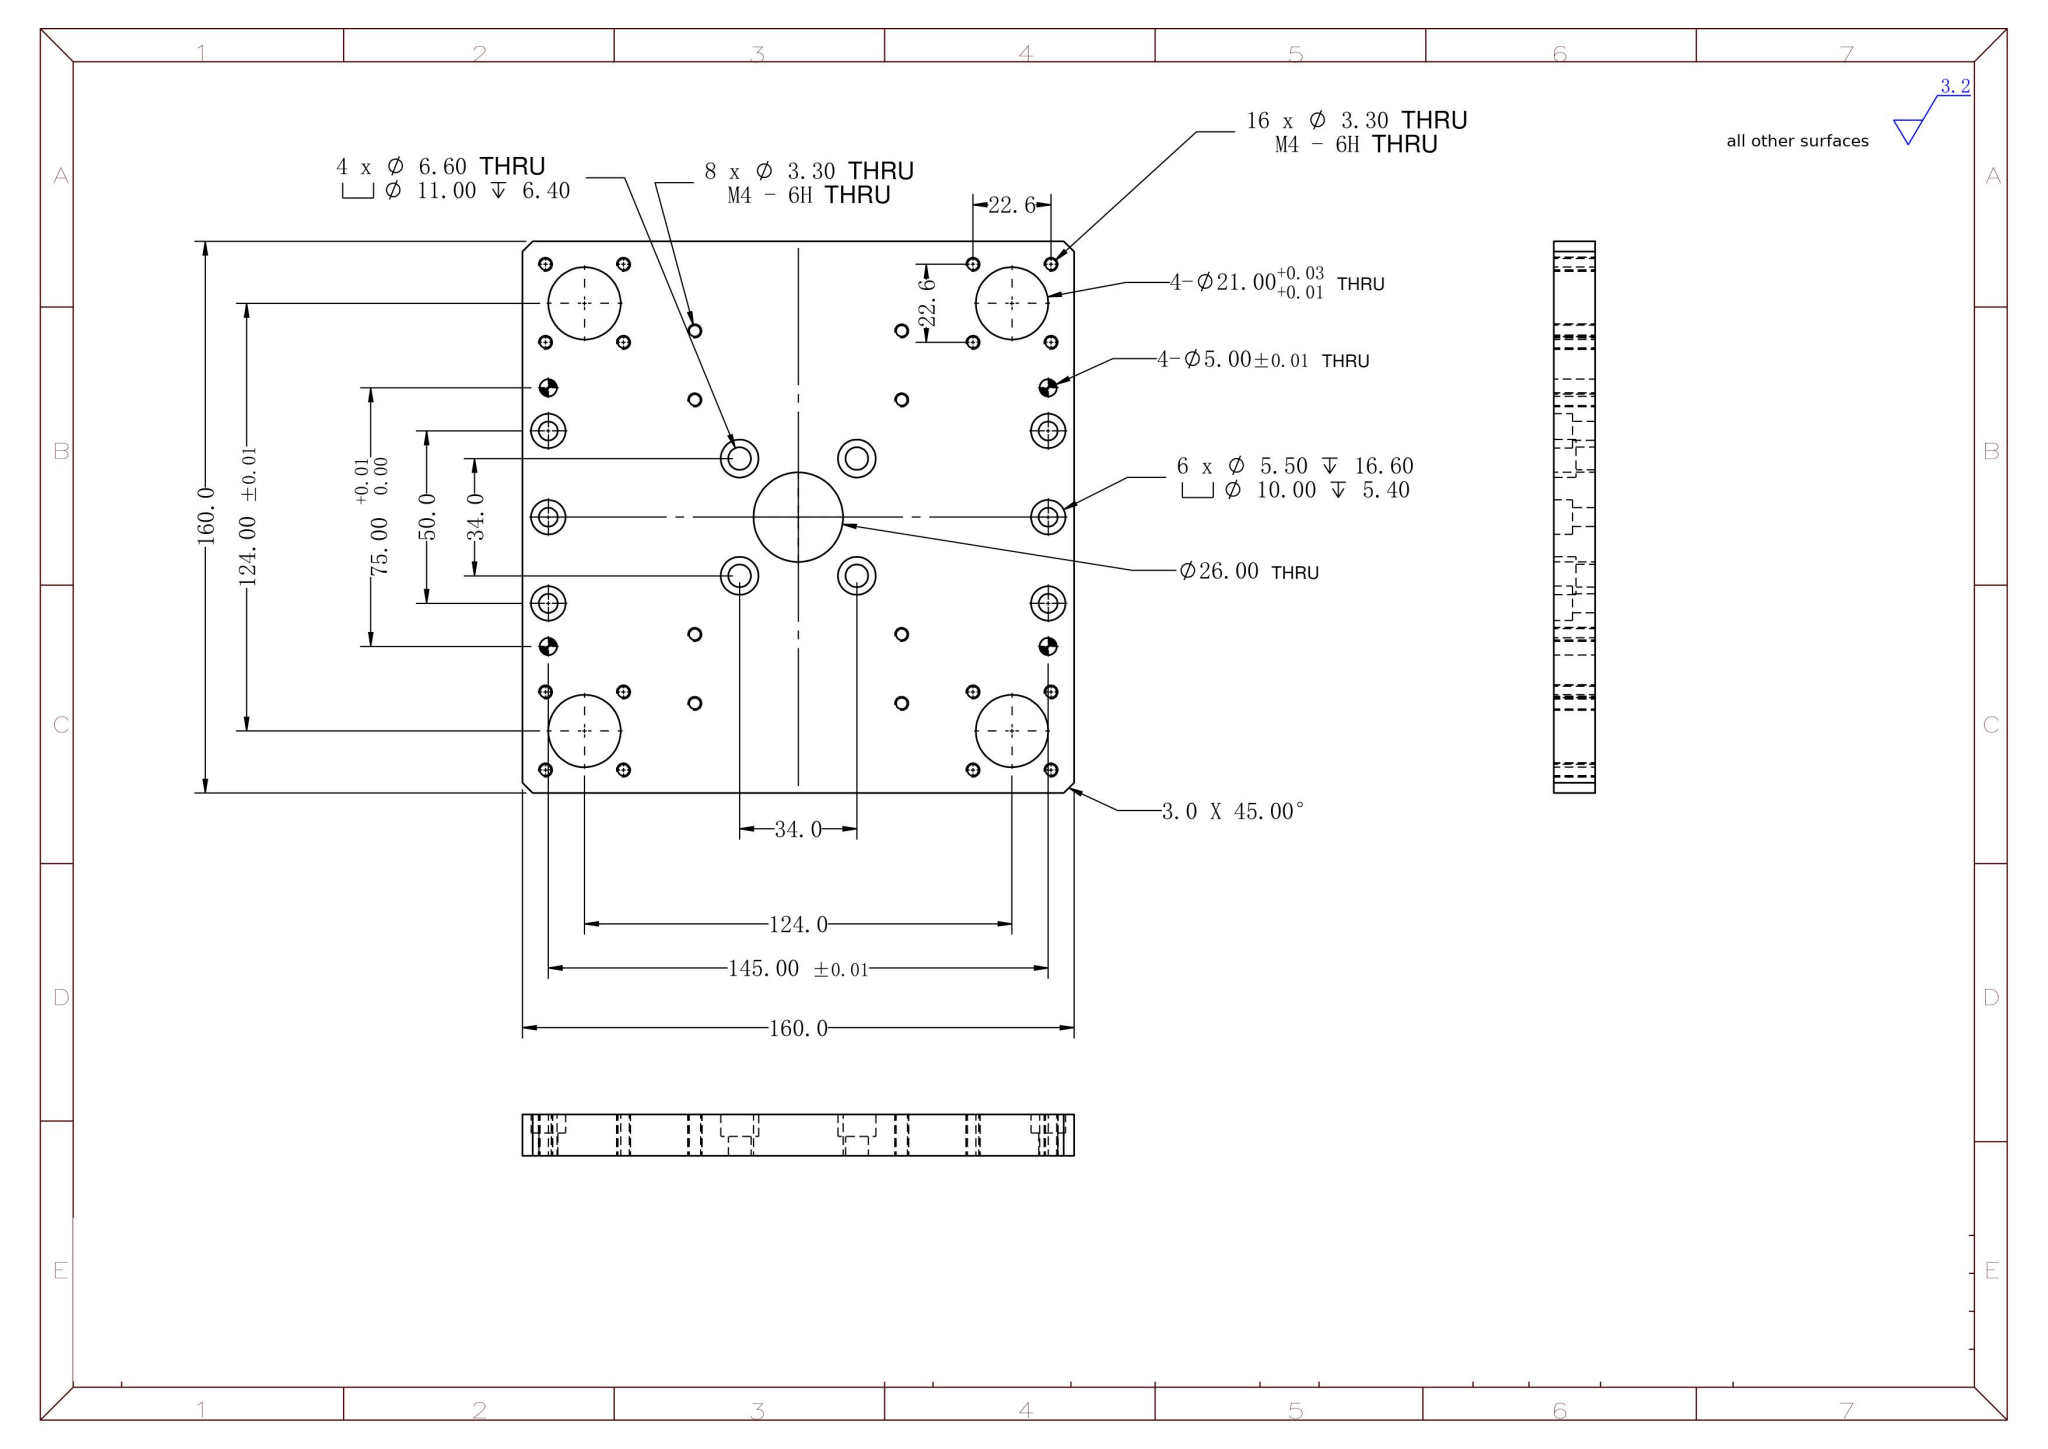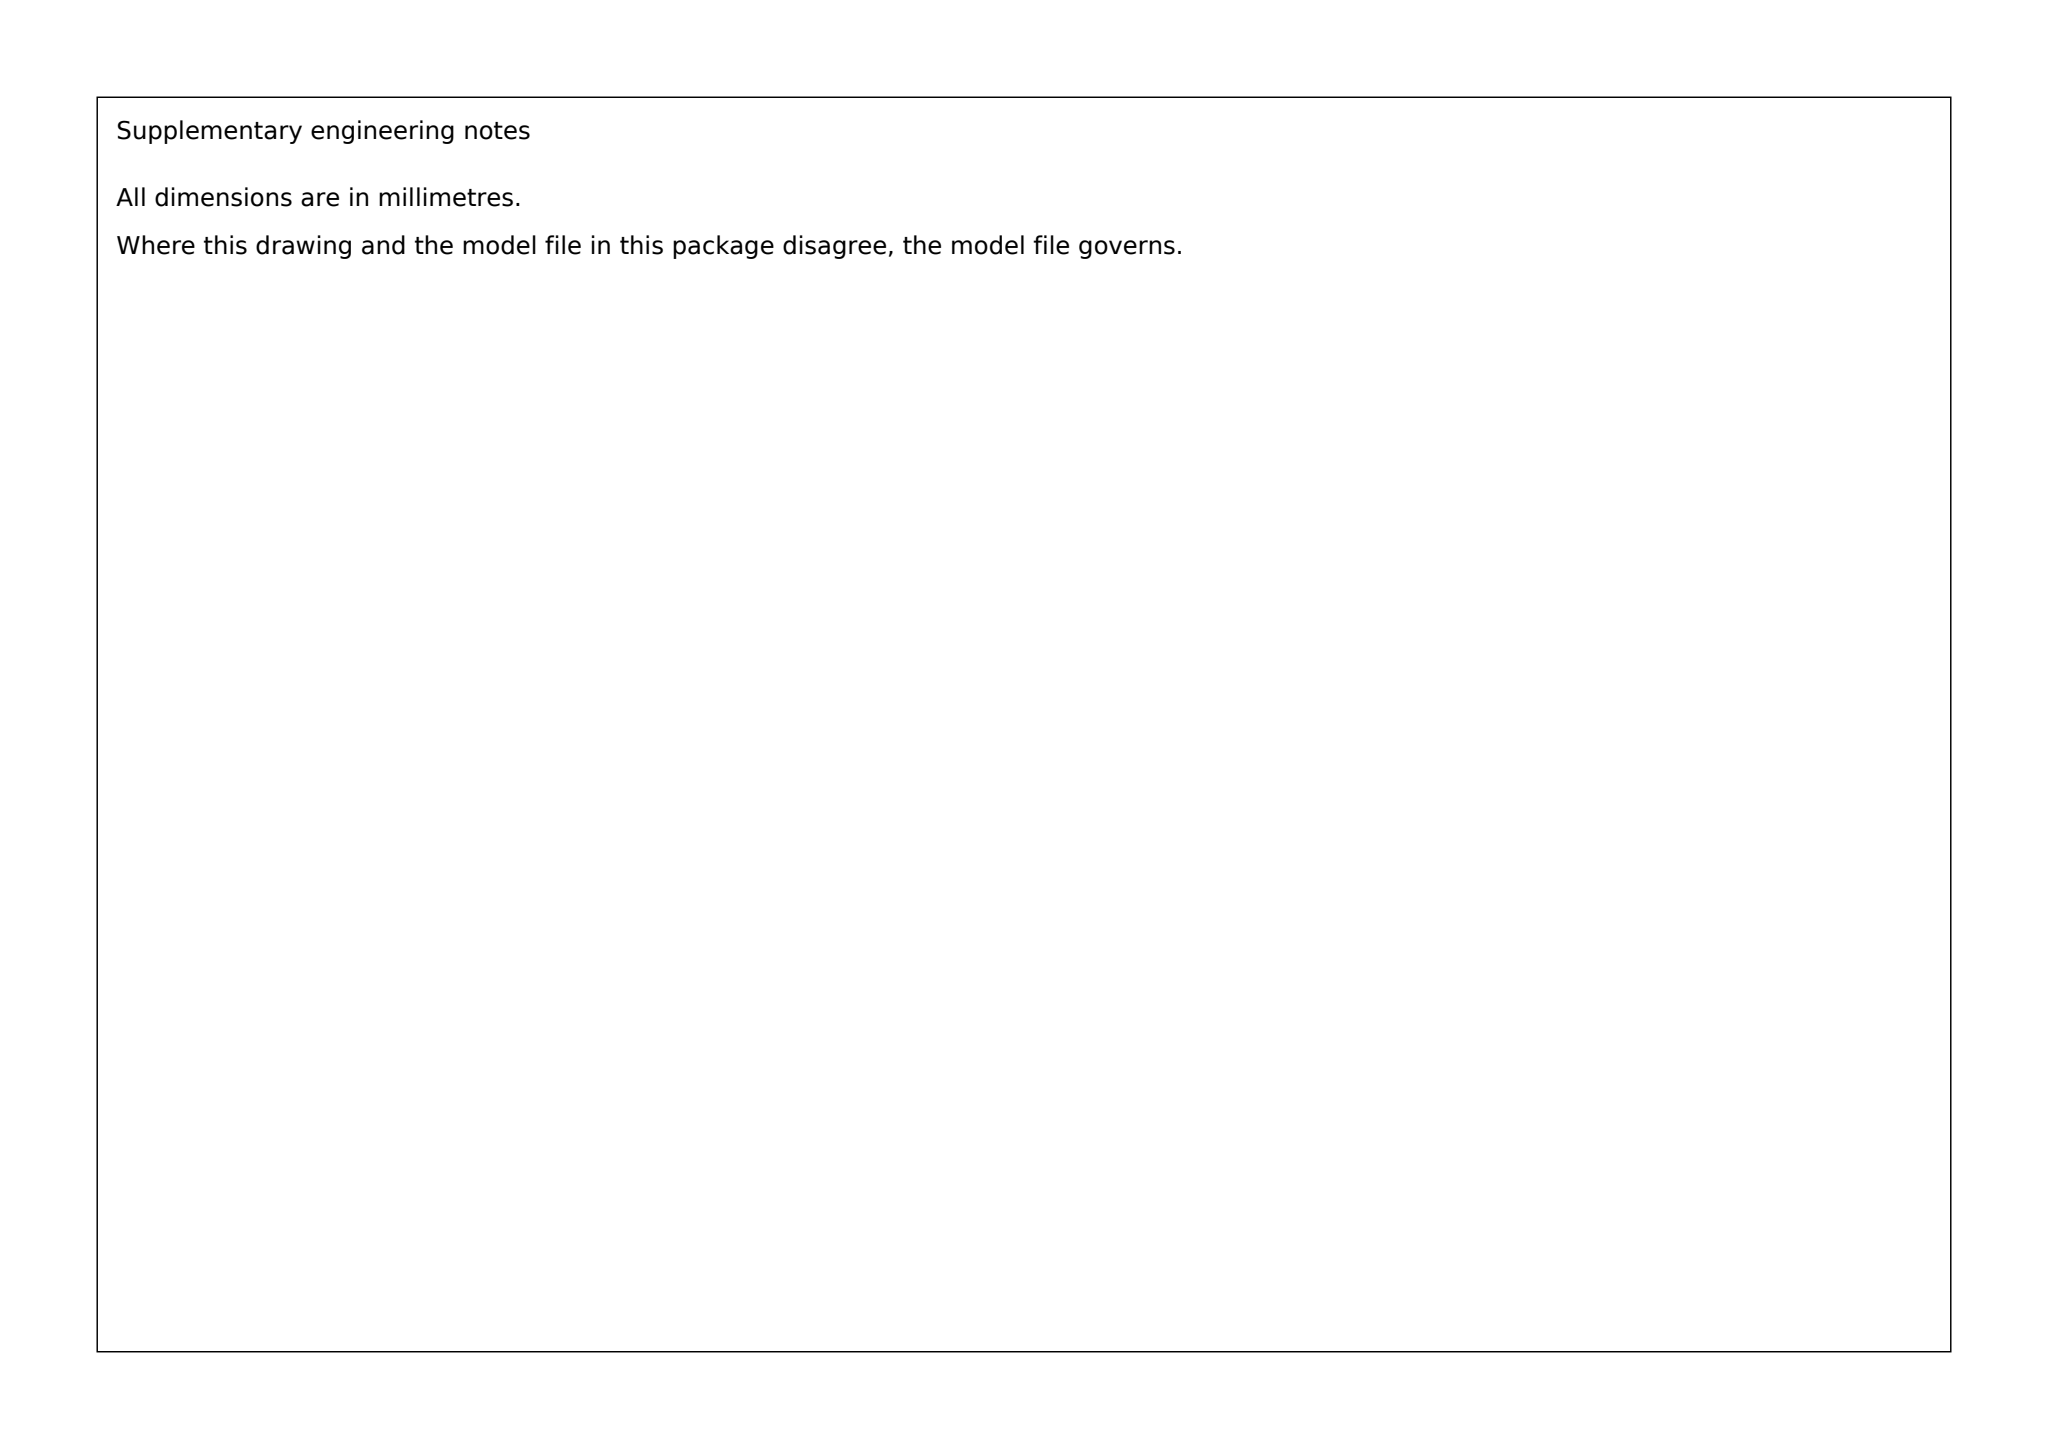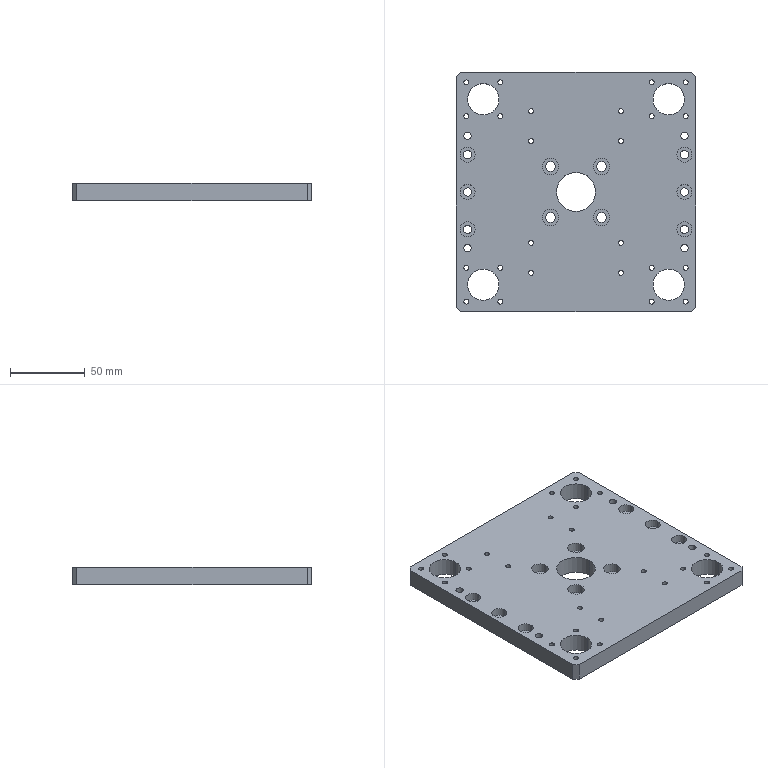Part | SolidWorks | mm | 1 solid | 126 faces | box 160 x 160 x 12 mm | volume 273897 mm3 | cylinder 106 | plane 20 | commonest cylinder face diameters 3.3 x48 10 x12 5.5 x12 5 x8 11 x8 6.6 x8 21 x8 26 x2
build123d program:
from build123d import *

# Parameters (mm, degrees)
SKETCH1_W                                       = 160
SKETCH1_H                                       = 160
BOSS_EXTRUDE1_DEPTH                             = 6
SKETCH2_R                                       = 10.5
CUT_EXTRUDE1_DEPTH                              = 114.772
M6_HEX_SOCKET_HEAD_CAP_SCREW_CBORE1_D           = 6.6
M6_HEX_SOCKET_HEAD_CAP_SCREW_CBORE1_CBORE_D     = 11
M6_HEX_SOCKET_HEAD_CAP_SCREW_CBORE1_CBORE_DEPTH = 6.4
SKETCH5_R                                       = 13
CUT_EXTRUDE2_DEPTH                              = 114.772
CHAMFER1_SIZE                                   = 3
M4_TAPPED_HOLE1_D                               = 3.3
CUT_EXTRUDE3_DEPTH                              = 114.772
CUT_EXTRUDE3_DEPTH_BACK                         = 114.772
SKETCH17_R                                      = 2.5
M5_HEX_SOCKET_HEAD_CAP_SCREW_CBORE1_D           = 5.5
M5_HEX_SOCKET_HEAD_CAP_SCREW_CBORE1_DEPTH       = 16.6
M5_HEX_SOCKET_HEAD_CAP_SCREW_CBORE1_CBORE_D     = 10
M5_HEX_SOCKET_HEAD_CAP_SCREW_CBORE1_CBORE_DEPTH = 5.4
M5_HEX_SOCKET_HEAD_CAP_SCREW_CBORE1_TIP         = 1.652
M4_TAPPED_HOLE2_D                               = 3.3


with BuildPart() as part:
    # Sketch1 → Boss-Extrude1 (new, symmetric)
    with BuildSketch(Plane.XY):
        Rectangle(SKETCH1_W, SKETCH1_H)
    extrude(amount=BOSS_EXTRUDE1_DEPTH, both=True)

    # Sketch2 → Cut-Extrude1 (cut, through all)
    with BuildSketch(Plane.XY.offset(6)):
        with Locations((-62, 62)):
            Circle(SKETCH2_R)
        with Locations((62, 62)):
            Circle(SKETCH2_R)
        with Locations((-62, -62)):
            Circle(SKETCH2_R)
        with Locations((62, -62)):
            Circle(SKETCH2_R)
    extrude(amount=-CUT_EXTRUDE1_DEPTH, mode=Mode.SUBTRACT)

    # M6 Hex Socket Head Cap Screw CBORE1 (through all)
    with Locations(Plane.XY.offset(6)):
        with Locations((-17, 17), (17, 17), (-17, -17), (17, -17)):
            CounterBoreHole(M6_HEX_SOCKET_HEAD_CAP_SCREW_CBORE1_D / 2, M6_HEX_SOCKET_HEAD_CAP_SCREW_CBORE1_CBORE_D / 2, M6_HEX_SOCKET_HEAD_CAP_SCREW_CBORE1_CBORE_DEPTH)

    # Sketch5 → Cut-Extrude2 (cut, through all)
    with BuildSketch(Plane.XY.offset(6)):
        Circle(SKETCH5_R)
    extrude(amount=-CUT_EXTRUDE2_DEPTH, mode=Mode.SUBTRACT)

    # Chamfer1
    chamfer1_edges = [part.edges().sort_by_distance(p)[0] for p in [
        (80, -80, 0),
        (-80, -80, 0),
        (-80, 80, 0),
        (80, 80, 0),
    ]]
    chamfer(chamfer1_edges, length=CHAMFER1_SIZE)

    # M4 Tapped Hole1 (through all)
    with Locations(Plane.XY.offset(6)):
        with Locations((-73.314, -73.314), (-50.686, -73.314), (-73.314, -50.686), (-50.686, -50.686), (73.314, -73.314), (50.686, -73.314), (50.686, -50.686), (73.314, -50.686), (73.314, 50.686), (50.686, 50.686), (50.686, 73.314), (73.314, 73.314), (-50.686, 50.686), (-73.314, 50.686), (-73.314, 73.314), (-50.686, 73.314)):
            Hole(M4_TAPPED_HOLE1_D / 2)

    # Sketch17 → Cut-Extrude3 (cut, two sides: drawn at the far end of the back side and taken through both)
    with BuildSketch(Plane(origin=(0, 0, -6), x_dir=(-1, 0, 0), z_dir=(0, 0, -1)).offset(-CUT_EXTRUDE3_DEPTH_BACK)):
        with Locations((-72.5, 37.5)):
            Circle(SKETCH17_R)
        with Locations((-72.5, -37.5)):
            Circle(SKETCH17_R)
        with Locations((72.5, -37.5)):
            Circle(SKETCH17_R)
        with Locations((72.5, 37.5)):
            Circle(SKETCH17_R)
    extrude(amount=CUT_EXTRUDE3_DEPTH + CUT_EXTRUDE3_DEPTH_BACK, mode=Mode.SUBTRACT)

    # M5 Hex Socket Head Cap Screw CBORE1
    with Locations(Plane.XY.offset(6)):
        with Locations((-72.5, 25), (-72.5, 0), (-72.5, -25), (72.5, 25), (72.5, 0), (72.5, -25)):
            CounterBoreHole(M5_HEX_SOCKET_HEAD_CAP_SCREW_CBORE1_D / 2, M5_HEX_SOCKET_HEAD_CAP_SCREW_CBORE1_CBORE_D / 2, M5_HEX_SOCKET_HEAD_CAP_SCREW_CBORE1_CBORE_DEPTH, depth=M5_HEX_SOCKET_HEAD_CAP_SCREW_CBORE1_DEPTH)
            with Locations((0, 0, -(M5_HEX_SOCKET_HEAD_CAP_SCREW_CBORE1_DEPTH + M5_HEX_SOCKET_HEAD_CAP_SCREW_CBORE1_TIP / 2))):  # 118° drill point
                Cone(0, M5_HEX_SOCKET_HEAD_CAP_SCREW_CBORE1_D / 2, M5_HEX_SOCKET_HEAD_CAP_SCREW_CBORE1_TIP, mode=Mode.SUBTRACT)

    # M4 Tapped Hole2 (through all)
    with Locations(Plane.XY.offset(6)):
        with Locations((30, 54), (30, 34), (30, -34), (30, -54), (-30, 54), (-30, 34), (-30, -34), (-30, -54)):
            Hole(M4_TAPPED_HOLE2_D / 2)


solid = part.part